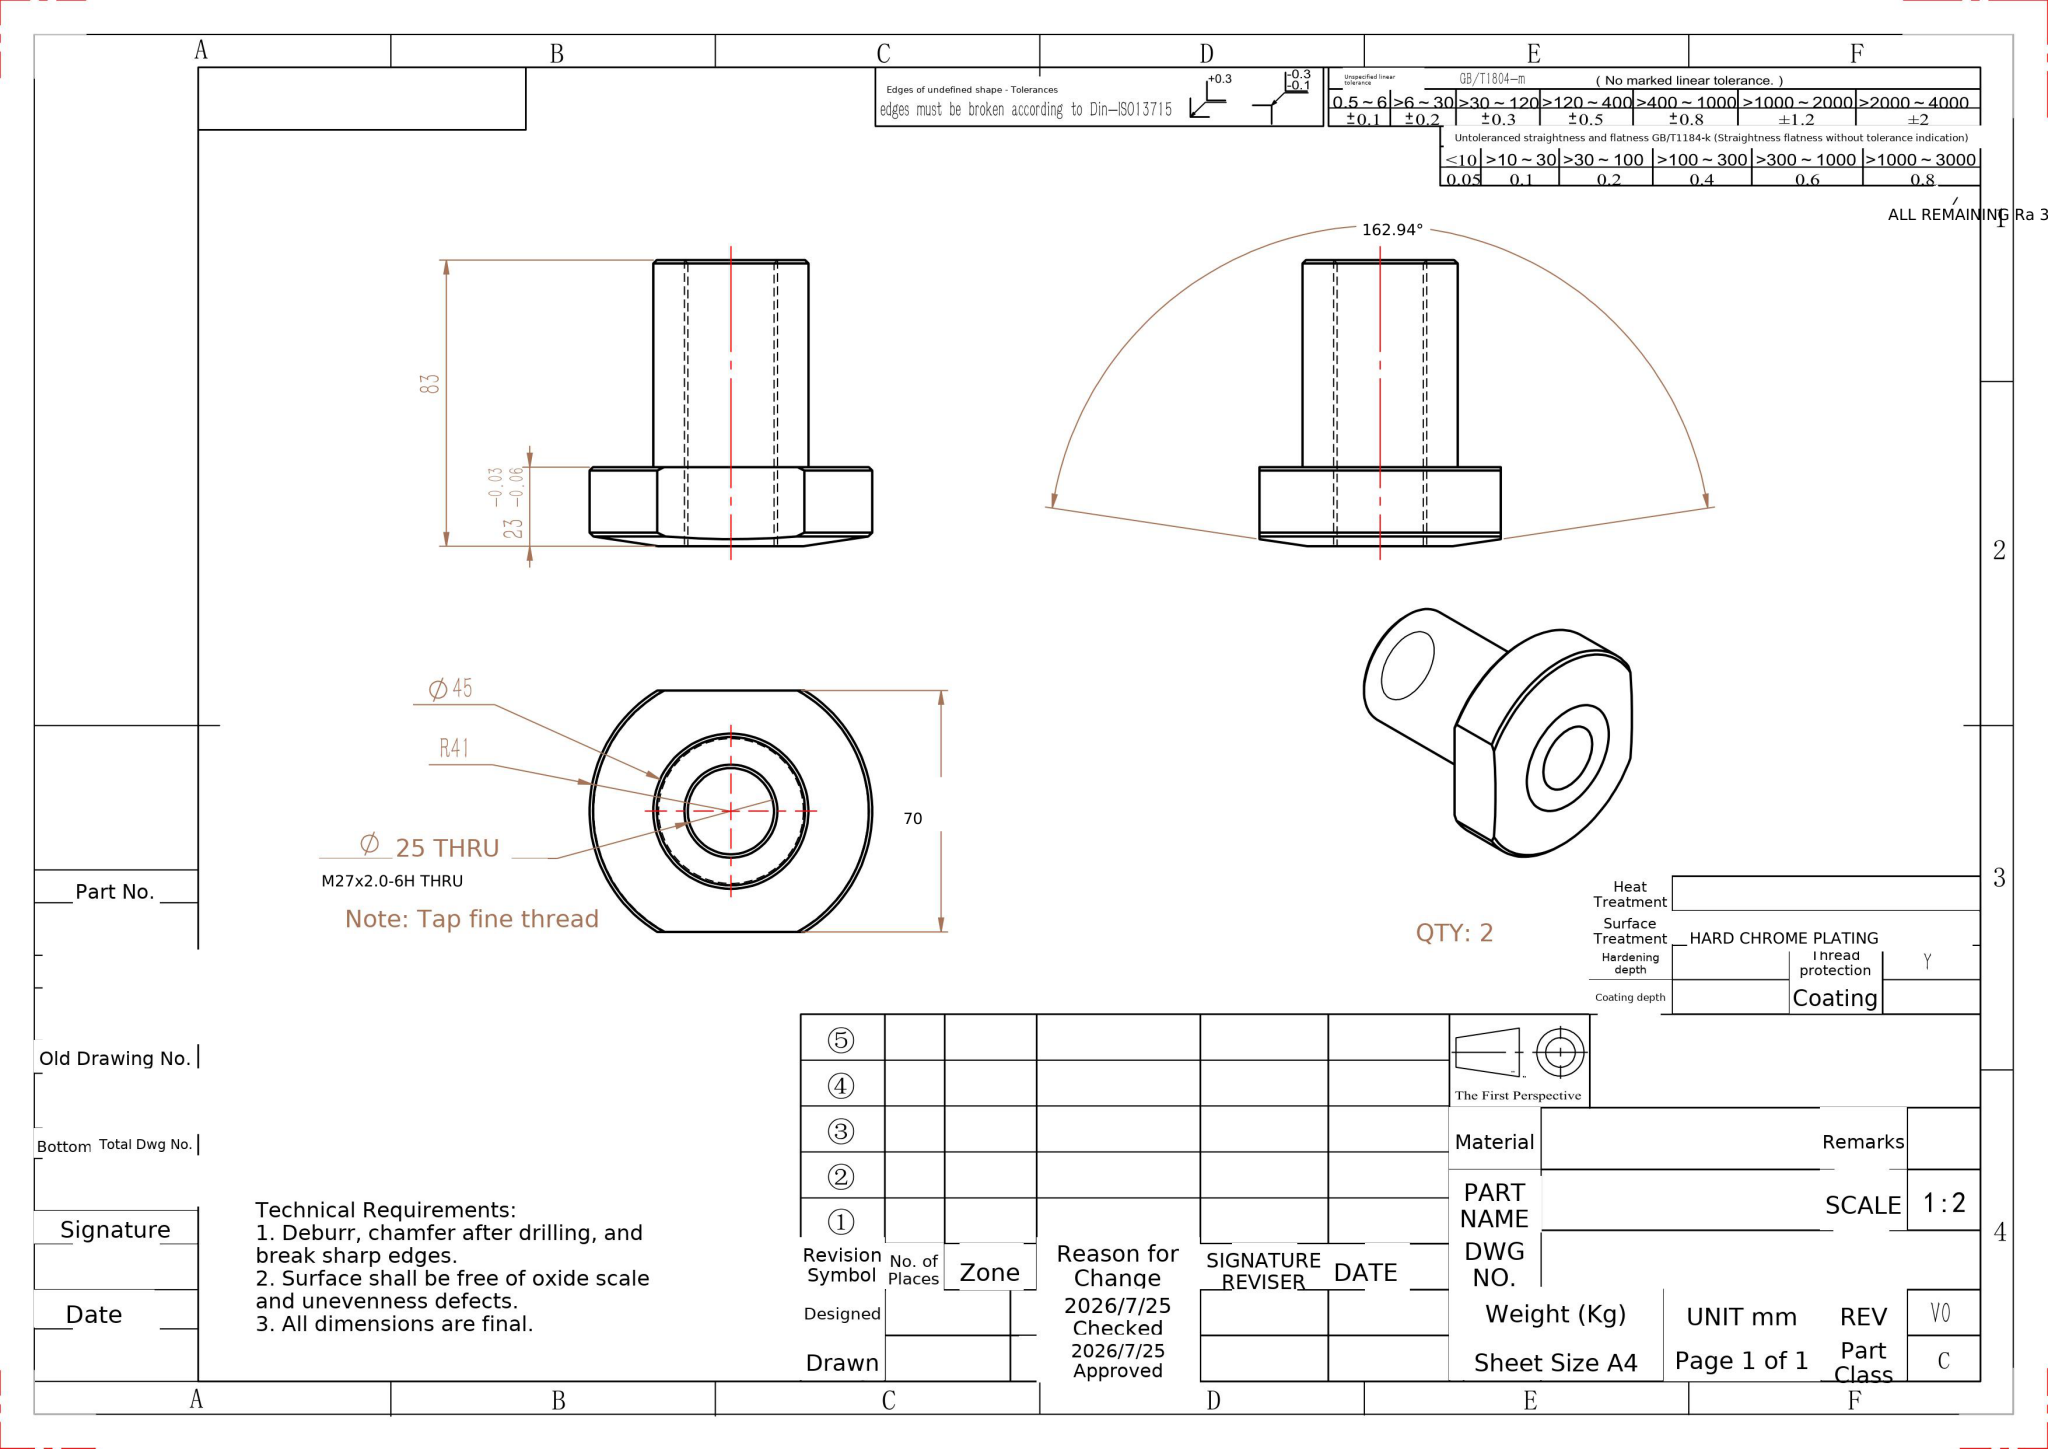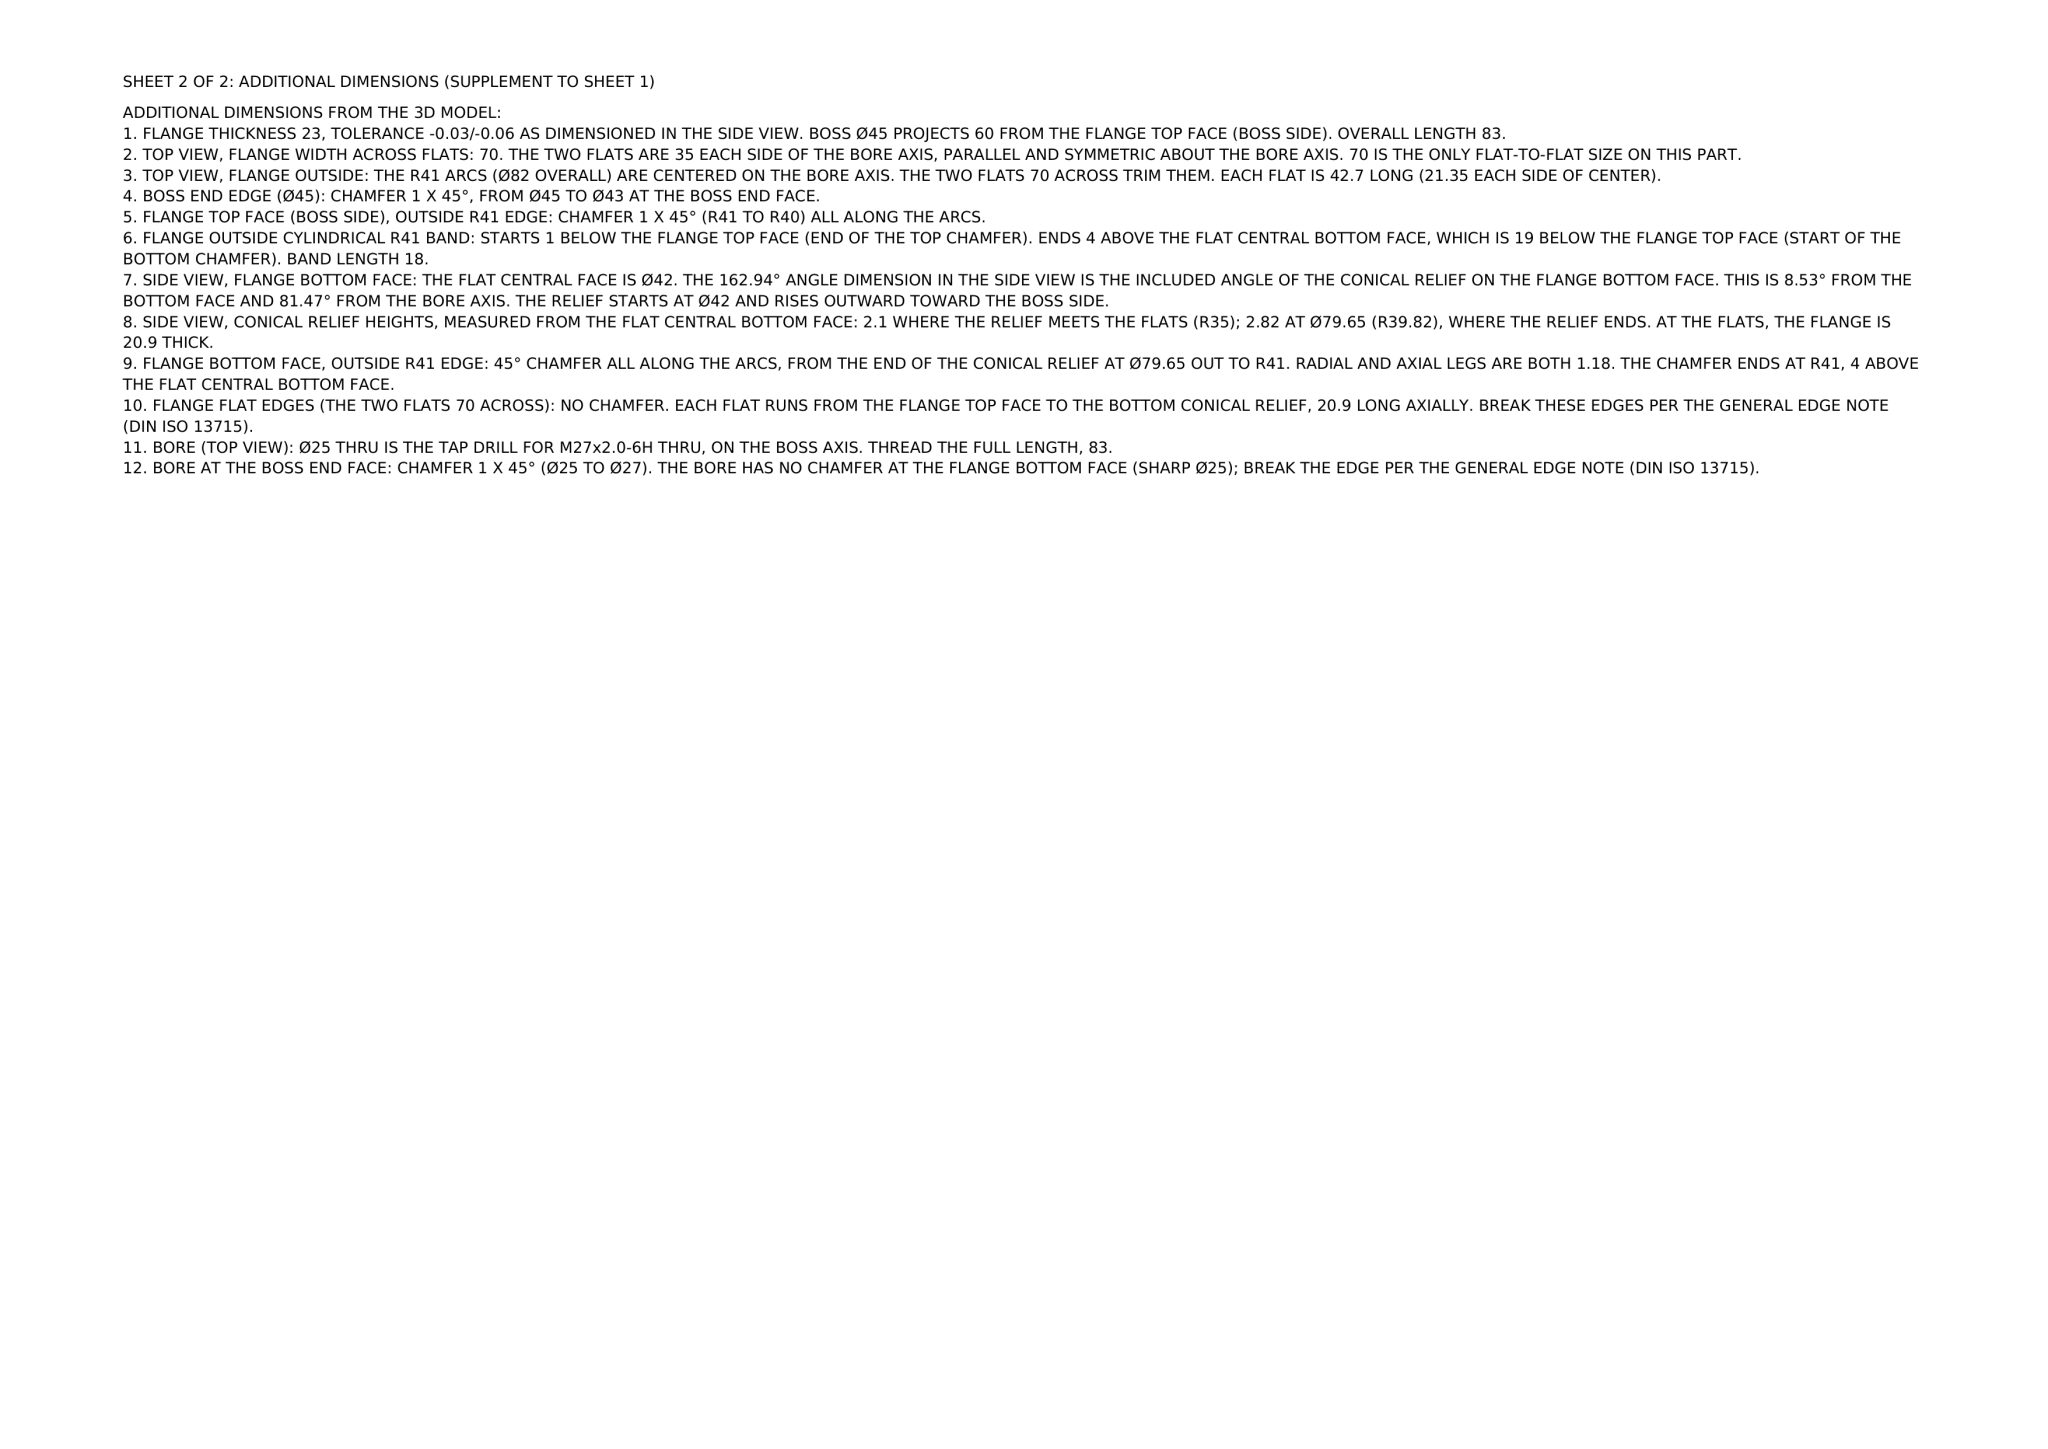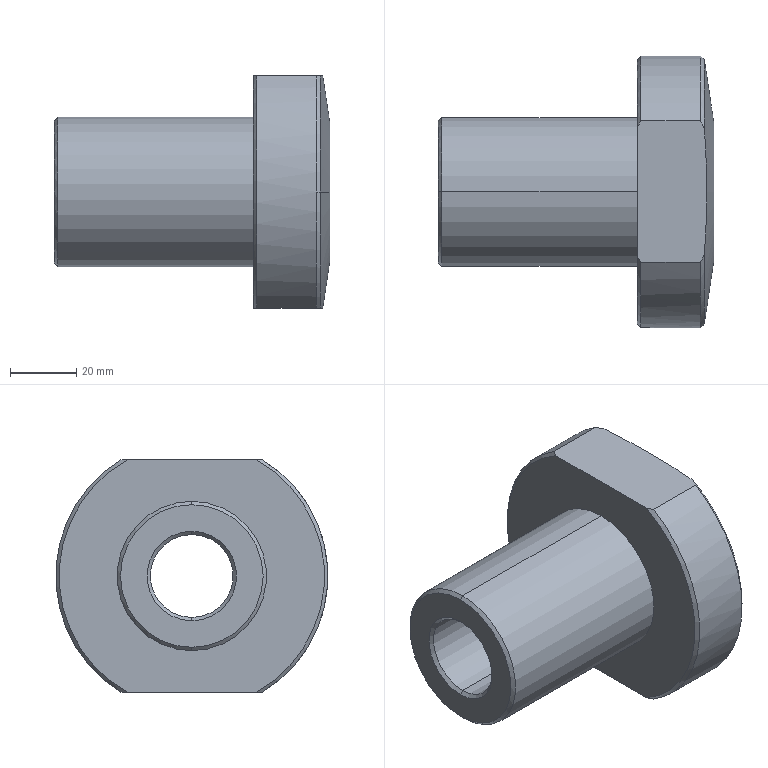Part | NX | mm | 1 solid | 22 faces | box 83 x 82 x 70 mm | volume 162318 mm3 | cone 11 | cylinder 6 | plane 5 | commonest cylinder face diameters 25 x2 45 x2 82 x2
STEP:
#1=CARTESIAN_POINT('',(23.176,-39.824,0.));
#2=VERTEX_POINT('',#1);
#3=CARTESIAN_POINT('',(23.176,-18.998,-35.));
#4=VERTEX_POINT('',#3);
#5=CARTESIAN_POINT('',(23.176,0.,0.));
#6=DIRECTION('',(1.,0.,0.));
#7=DIRECTION('',(-0.,1.,0.));
#8=AXIS2_PLACEMENT_3D('',#5,#6,#7);
#9=CIRCLE('',#8,39.824);
#10=EDGE_CURVE('',#2,#4,#9,.T.);
#11=ORIENTED_EDGE('',*,*,#10,.F.);
#12=CARTESIAN_POINT('',(22.,-41.,0.));
#13=VERTEX_POINT('',#12);
#14=CARTESIAN_POINT('',(23.176,-39.824,0.));
#15=DIRECTION('',(-0.7071,-0.7071,0.));
#16=VECTOR('',#15,1000.);
#17=LINE('',#14,#16);
#18=EDGE_CURVE('',#2,#13,#17,.T.);
#19=ORIENTED_EDGE('',*,*,#18,.T.);
#20=CARTESIAN_POINT('',(22.,-21.354,-35.));
#21=VERTEX_POINT('',#20);
#22=CARTESIAN_POINT('',(22.,0.,0.));
#23=DIRECTION('',(-1.,-0.,0.));
#24=DIRECTION('',(-0.,1.,0.));
#25=AXIS2_PLACEMENT_3D('',#22,#23,#24);
#26=CIRCLE('',#25,41.);
#27=EDGE_CURVE('',#21,#13,#26,.T.);
#28=ORIENTED_EDGE('',*,*,#27,.F.);
#29=CARTESIAN_POINT('',(23.176,-18.998,-35.));
#30=CARTESIAN_POINT('',(22.798,-19.79,-35.));
#31=CARTESIAN_POINT('',(22.406,-20.575,-35.));
#32=CARTESIAN_POINT('',(22.,-21.354,-35.));
#33=B_SPLINE_CURVE_WITH_KNOTS('',3,(#29,#30,#31,#32),.UNSPECIFIED.,.F.,.F.,(4,4),(0.,0.002634),.UNSPECIFIED.);
#34=EDGE_CURVE('',#4,#21,#33,.T.);
#35=ORIENTED_EDGE('',*,*,#34,.F.);
#36=EDGE_LOOP('',(#11,#19,#28,#35));
#37=FACE_OUTER_BOUND('',#36,.T.);
#38=CARTESIAN_POINT('',(23.176,0.,0.));
#39=DIRECTION('',(-1.,-0.,0.));
#40=DIRECTION('',(0.,-1.,0.));
#41=AXIS2_PLACEMENT_3D('',#38,#39,#40);
#42=CONICAL_SURFACE('',#41,39.824,0.7854);
#43=ADVANCED_FACE('',(#37),#42,.T.);
#44=CARTESIAN_POINT('',(-57.,0.,21.5));
#45=VERTEX_POINT('',#44);
#46=CARTESIAN_POINT('',(-57.,0.,-21.5));
#47=VERTEX_POINT('',#46);
#48=CARTESIAN_POINT('',(-57.,0.,0.));
#49=DIRECTION('',(-1.,0.,0.));
#50=DIRECTION('',(0.,0.,1.));
#51=AXIS2_PLACEMENT_3D('',#48,#49,#50);
#52=CIRCLE('',#51,21.5);
#53=EDGE_CURVE('',#45,#47,#52,.T.);
#54=ORIENTED_EDGE('',*,*,#53,.F.);
#55=CARTESIAN_POINT('',(-56.,0.,22.5));
#56=VERTEX_POINT('',#55);
#57=CARTESIAN_POINT('',(-57.,0.,21.5));
#58=DIRECTION('',(0.7071,0.,0.7071));
#59=VECTOR('',#58,1000.);
#60=LINE('',#57,#59);
#61=EDGE_CURVE('',#45,#56,#60,.T.);
#62=ORIENTED_EDGE('',*,*,#61,.T.);
#63=CARTESIAN_POINT('',(-56.,0.,-22.5));
#64=VERTEX_POINT('',#63);
#65=CARTESIAN_POINT('',(-56.,0.,0.));
#66=DIRECTION('',(1.,0.,0.));
#67=DIRECTION('',(0.,0.,1.));
#68=AXIS2_PLACEMENT_3D('',#65,#66,#67);
#69=CIRCLE('',#68,22.5);
#70=EDGE_CURVE('',#64,#56,#69,.T.);
#71=ORIENTED_EDGE('',*,*,#70,.F.);
#72=CARTESIAN_POINT('',(-57.,0.,-21.5));
#73=DIRECTION('',(0.7071,0.,-0.7071));
#74=VECTOR('',#73,1000.);
#75=LINE('',#72,#74);
#76=EDGE_CURVE('',#47,#64,#75,.T.);
#77=ORIENTED_EDGE('',*,*,#76,.F.);
#78=EDGE_LOOP('',(#54,#62,#71,#77));
#79=FACE_OUTER_BOUND('',#78,.T.);
#80=CARTESIAN_POINT('',(-57.,0.,0.));
#81=DIRECTION('',(1.,0.,0.));
#82=DIRECTION('',(0.,0.,-1.));
#83=AXIS2_PLACEMENT_3D('',#80,#81,#82);
#84=CONICAL_SURFACE('',#83,21.5,0.7854);
#85=ADVANCED_FACE('',(#79),#84,.T.);
#86=CARTESIAN_POINT('',(-56.,0.,-12.5));
#87=VERTEX_POINT('',#86);
#88=CARTESIAN_POINT('',(-56.,0.,12.5));
#89=VERTEX_POINT('',#88);
#90=CARTESIAN_POINT('',(-56.,0.,0.));
#91=DIRECTION('',(-1.,0.,0.));
#92=DIRECTION('',(0.,0.,1.));
#93=AXIS2_PLACEMENT_3D('',#90,#91,#92);
#94=CIRCLE('',#93,12.5);
#95=EDGE_CURVE('',#87,#89,#94,.T.);
#96=ORIENTED_EDGE('',*,*,#95,.F.);
#97=CARTESIAN_POINT('',(-57.,0.,-13.5));
#98=VERTEX_POINT('',#97);
#99=CARTESIAN_POINT('',(-56.,0.,-12.5));
#100=DIRECTION('',(-0.7071,0.,-0.7071));
#101=VECTOR('',#100,1000.);
#102=LINE('',#99,#101);
#103=EDGE_CURVE('',#87,#98,#102,.T.);
#104=ORIENTED_EDGE('',*,*,#103,.T.);
#105=CARTESIAN_POINT('',(-57.,0.,13.5));
#106=VERTEX_POINT('',#105);
#107=CARTESIAN_POINT('',(-57.,0.,0.));
#108=DIRECTION('',(1.,0.,0.));
#109=DIRECTION('',(0.,0.,1.));
#110=AXIS2_PLACEMENT_3D('',#107,#108,#109);
#111=CIRCLE('',#110,13.5);
#112=EDGE_CURVE('',#106,#98,#111,.T.);
#113=ORIENTED_EDGE('',*,*,#112,.F.);
#114=CARTESIAN_POINT('',(-56.,0.,12.5));
#115=DIRECTION('',(-0.7071,0.,0.7071));
#116=VECTOR('',#115,1000.);
#117=LINE('',#114,#116);
#118=EDGE_CURVE('',#89,#106,#117,.T.);
#119=ORIENTED_EDGE('',*,*,#118,.F.);
#120=EDGE_LOOP('',(#96,#104,#113,#119));
#121=FACE_OUTER_BOUND('',#120,.T.);
#122=CARTESIAN_POINT('',(-56.,0.,0.));
#123=DIRECTION('',(-1.,0.,0.));
#124=DIRECTION('',(0.,0.,1.));
#125=AXIS2_PLACEMENT_3D('',#122,#123,#124);
#126=CONICAL_SURFACE('',#125,12.5,0.7854);
#127=ADVANCED_FACE('',(#121),#126,.F.);
#128=CARTESIAN_POINT('',(26.,0.,-12.5));
#129=VERTEX_POINT('',#128);
#130=CARTESIAN_POINT('',(26.,0.,12.5));
#131=VERTEX_POINT('',#130);
#132=CARTESIAN_POINT('',(26.,0.,0.));
#133=DIRECTION('',(-1.,0.,0.));
#134=DIRECTION('',(0.,0.,1.));
#135=AXIS2_PLACEMENT_3D('',#132,#133,#134);
#136=CIRCLE('',#135,12.5);
#137=EDGE_CURVE('',#129,#131,#136,.T.);
#138=ORIENTED_EDGE('',*,*,#137,.F.);
#139=CARTESIAN_POINT('',(-57.,0.,-12.5));
#140=DIRECTION('',(-1.,0.,0.));
#141=VECTOR('',#140,1000.);
#142=LINE('',#139,#141);
#143=EDGE_CURVE('',#129,#87,#142,.T.);
#144=ORIENTED_EDGE('',*,*,#143,.T.);
#145=ORIENTED_EDGE('',*,*,#95,.T.);
#146=CARTESIAN_POINT('',(-57.,0.,12.5));
#147=DIRECTION('',(-1.,0.,0.));
#148=VECTOR('',#147,1000.);
#149=LINE('',#146,#148);
#150=EDGE_CURVE('',#131,#89,#149,.T.);
#151=ORIENTED_EDGE('',*,*,#150,.F.);
#152=EDGE_LOOP('',(#138,#144,#145,#151));
#153=FACE_OUTER_BOUND('',#152,.T.);
#154=CARTESIAN_POINT('',(-57.,0.,0.));
#155=DIRECTION('',(-1.,0.,0.));
#156=DIRECTION('',(0.,0.,1.));
#157=AXIS2_PLACEMENT_3D('',#154,#155,#156);
#158=CYLINDRICAL_SURFACE('',#157,12.5);
#159=ADVANCED_FACE('',(#153),#158,.F.);
#160=ORIENTED_EDGE('',*,*,#70,.T.);
#161=CARTESIAN_POINT('',(3.,0.,22.5));
#162=VERTEX_POINT('',#161);
#163=CARTESIAN_POINT('',(-57.,0.,22.5));
#164=DIRECTION('',(1.,0.,0.));
#165=VECTOR('',#164,1000.);
#166=LINE('',#163,#165);
#167=EDGE_CURVE('',#56,#162,#166,.T.);
#168=ORIENTED_EDGE('',*,*,#167,.T.);
#169=CARTESIAN_POINT('',(3.,0.,-22.5));
#170=VERTEX_POINT('',#169);
#171=CARTESIAN_POINT('',(3.,0.,0.));
#172=DIRECTION('',(-1.,0.,0.));
#173=DIRECTION('',(0.,0.,1.));
#174=AXIS2_PLACEMENT_3D('',#171,#172,#173);
#175=CIRCLE('',#174,22.5);
#176=EDGE_CURVE('',#162,#170,#175,.T.);
#177=ORIENTED_EDGE('',*,*,#176,.T.);
#178=CARTESIAN_POINT('',(-57.,0.,-22.5));
#179=DIRECTION('',(1.,0.,0.));
#180=VECTOR('',#179,1000.);
#181=LINE('',#178,#180);
#182=EDGE_CURVE('',#64,#170,#181,.T.);
#183=ORIENTED_EDGE('',*,*,#182,.F.);
#184=EDGE_LOOP('',(#160,#168,#177,#183));
#185=FACE_OUTER_BOUND('',#184,.T.);
#186=CARTESIAN_POINT('',(-57.,0.,0.));
#187=DIRECTION('',(1.,0.,0.));
#188=DIRECTION('',(0.,0.,-1.));
#189=AXIS2_PLACEMENT_3D('',#186,#187,#188);
#190=CYLINDRICAL_SURFACE('',#189,22.5);
#191=ADVANCED_FACE('',(#185),#190,.T.);
#192=CARTESIAN_POINT('',(26.,21.,0.));
#193=VERTEX_POINT('',#192);
#194=CARTESIAN_POINT('',(26.,-21.,0.));
#195=VERTEX_POINT('',#194);
#196=CARTESIAN_POINT('',(26.,0.,0.));
#197=DIRECTION('',(1.,0.,0.));
#198=DIRECTION('',(-0.,1.,0.));
#199=AXIS2_PLACEMENT_3D('',#196,#197,#198);
#200=CIRCLE('',#199,21.);
#201=EDGE_CURVE('',#193,#195,#200,.T.);
#202=ORIENTED_EDGE('',*,*,#201,.F.);
#203=CARTESIAN_POINT('',(23.176,39.824,0.));
#204=VERTEX_POINT('',#203);
#205=CARTESIAN_POINT('',(26.,21.,0.));
#206=DIRECTION('',(-0.1483,0.9889,0.));
#207=VECTOR('',#206,1000.);
#208=LINE('',#205,#207);
#209=EDGE_CURVE('',#193,#204,#208,.T.);
#210=ORIENTED_EDGE('',*,*,#209,.T.);
#211=CARTESIAN_POINT('',(23.176,18.998,35.));
#212=VERTEX_POINT('',#211);
#213=CARTESIAN_POINT('',(23.176,0.,0.));
#214=DIRECTION('',(1.,0.,0.));
#215=DIRECTION('',(-0.,1.,0.));
#216=AXIS2_PLACEMENT_3D('',#213,#214,#215);
#217=CIRCLE('',#216,39.824);
#218=EDGE_CURVE('',#204,#212,#217,.T.);
#219=ORIENTED_EDGE('',*,*,#218,.T.);
#220=CARTESIAN_POINT('',(23.176,-18.998,35.));
#221=VERTEX_POINT('',#220);
#222=CARTESIAN_POINT('',(23.176,18.998,35.));
#223=CARTESIAN_POINT('',(23.402,15.846,35.));
#224=CARTESIAN_POINT('',(23.584,12.691,35.));
#225=CARTESIAN_POINT('',(23.833,6.372,35.));
#226=CARTESIAN_POINT('',(23.899,3.208,35.));
#227=CARTESIAN_POINT('',(23.901,-3.129,35.));
#228=CARTESIAN_POINT('',(23.835,-6.303,35.));
#229=CARTESIAN_POINT('',(23.586,-12.659,35.));
#230=CARTESIAN_POINT('',(23.403,-15.83,35.));
#231=CARTESIAN_POINT('',(23.176,-18.998,35.));
#232=B_SPLINE_CURVE_WITH_KNOTS('',3,(#222,#223,#224,#225,#226,#227,#228,#229,#230,#231),.UNSPECIFIED.,.F.,.F.,(4,2,2,2,4),(0.04542,0.0549,0.06438,0.07386,0.08334),.UNSPECIFIED.);
#233=EDGE_CURVE('',#212,#221,#232,.T.);
#234=ORIENTED_EDGE('',*,*,#233,.T.);
#235=CARTESIAN_POINT('',(23.176,0.,0.));
#236=DIRECTION('',(1.,0.,0.));
#237=DIRECTION('',(-0.,1.,0.));
#238=AXIS2_PLACEMENT_3D('',#235,#236,#237);
#239=CIRCLE('',#238,39.824);
#240=EDGE_CURVE('',#221,#2,#239,.T.);
#241=ORIENTED_EDGE('',*,*,#240,.T.);
#242=CARTESIAN_POINT('',(26.,-21.,0.));
#243=DIRECTION('',(-0.1483,-0.9889,0.));
#244=VECTOR('',#243,1000.);
#245=LINE('',#242,#244);
#246=EDGE_CURVE('',#195,#2,#245,.T.);
#247=ORIENTED_EDGE('',*,*,#246,.F.);
#248=EDGE_LOOP('',(#202,#210,#219,#234,#241,#247));
#249=FACE_OUTER_BOUND('',#248,.T.);
#250=CARTESIAN_POINT('',(26.,0.,0.));
#251=DIRECTION('',(-1.,-0.,0.));
#252=DIRECTION('',(0.,-1.,0.));
#253=AXIS2_PLACEMENT_3D('',#250,#251,#252);
#254=CONICAL_SURFACE('',#253,21.,1.422);
#255=ADVANCED_FACE('',(#249),#254,.T.);
#256=CARTESIAN_POINT('',(22.,21.354,35.));
#257=VERTEX_POINT('',#256);
#258=CARTESIAN_POINT('',(4.,21.354,35.));
#259=VERTEX_POINT('',#258);
#260=CARTESIAN_POINT('',(141.966,21.354,35.));
#261=DIRECTION('',(-1.,0.,0.));
#262=VECTOR('',#261,1000.);
#263=LINE('',#260,#262);
#264=EDGE_CURVE('',#257,#259,#263,.T.);
#265=ORIENTED_EDGE('',*,*,#264,.F.);
#266=CARTESIAN_POINT('',(22.,21.354,-35.));
#267=VERTEX_POINT('',#266);
#268=CARTESIAN_POINT('',(22.,0.,0.));
#269=DIRECTION('',(-1.,-0.,0.));
#270=DIRECTION('',(-0.,1.,0.));
#271=AXIS2_PLACEMENT_3D('',#268,#269,#270);
#272=CIRCLE('',#271,41.);
#273=EDGE_CURVE('',#257,#267,#272,.T.);
#274=ORIENTED_EDGE('',*,*,#273,.T.);
#275=CARTESIAN_POINT('',(4.,21.354,-35.));
#276=VERTEX_POINT('',#275);
#277=CARTESIAN_POINT('',(141.966,21.354,-35.));
#278=DIRECTION('',(1.,0.,0.));
#279=VECTOR('',#278,1000.);
#280=LINE('',#277,#279);
#281=EDGE_CURVE('',#276,#267,#280,.T.);
#282=ORIENTED_EDGE('',*,*,#281,.F.);
#283=CARTESIAN_POINT('',(4.,0.,0.));
#284=DIRECTION('',(1.,0.,0.));
#285=DIRECTION('',(0.,-0.,1.));
#286=AXIS2_PLACEMENT_3D('',#283,#284,#285);
#287=CIRCLE('',#286,41.);
#288=EDGE_CURVE('',#276,#259,#287,.T.);
#289=ORIENTED_EDGE('',*,*,#288,.T.);
#290=EDGE_LOOP('',(#265,#274,#282,#289));
#291=FACE_OUTER_BOUND('',#290,.T.);
#292=CARTESIAN_POINT('',(141.966,0.,0.));
#293=DIRECTION('',(-1.,0.,0.));
#294=DIRECTION('',(0.,0.,1.));
#295=AXIS2_PLACEMENT_3D('',#292,#293,#294);
#296=CYLINDRICAL_SURFACE('',#295,41.);
#297=ADVANCED_FACE('',(#291),#296,.T.);
#298=CARTESIAN_POINT('',(4.,-21.354,-35.));
#299=VERTEX_POINT('',#298);
#300=CARTESIAN_POINT('',(141.966,-21.354,-35.));
#301=DIRECTION('',(-1.,0.,0.));
#302=VECTOR('',#301,1000.);
#303=LINE('',#300,#302);
#304=EDGE_CURVE('',#21,#299,#303,.T.);
#305=ORIENTED_EDGE('',*,*,#304,.F.);
#306=ORIENTED_EDGE('',*,*,#27,.T.);
#307=CARTESIAN_POINT('',(22.,-21.354,35.));
#308=VERTEX_POINT('',#307);
#309=CARTESIAN_POINT('',(22.,0.,0.));
#310=DIRECTION('',(-1.,-0.,0.));
#311=DIRECTION('',(-0.,1.,0.));
#312=AXIS2_PLACEMENT_3D('',#309,#310,#311);
#313=CIRCLE('',#312,41.);
#314=EDGE_CURVE('',#13,#308,#313,.T.);
#315=ORIENTED_EDGE('',*,*,#314,.T.);
#316=CARTESIAN_POINT('',(4.,-21.354,35.));
#317=VERTEX_POINT('',#316);
#318=CARTESIAN_POINT('',(141.966,-21.354,35.));
#319=DIRECTION('',(1.,0.,0.));
#320=VECTOR('',#319,1000.);
#321=LINE('',#318,#320);
#322=EDGE_CURVE('',#317,#308,#321,.T.);
#323=ORIENTED_EDGE('',*,*,#322,.F.);
#324=CARTESIAN_POINT('',(4.,0.,0.));
#325=DIRECTION('',(1.,0.,0.));
#326=DIRECTION('',(0.,0.,1.));
#327=AXIS2_PLACEMENT_3D('',#324,#325,#326);
#328=CIRCLE('',#327,41.);
#329=EDGE_CURVE('',#317,#299,#328,.T.);
#330=ORIENTED_EDGE('',*,*,#329,.T.);
#331=EDGE_LOOP('',(#305,#306,#315,#323,#330));
#332=FACE_OUTER_BOUND('',#331,.T.);
#333=CARTESIAN_POINT('',(141.966,0.,0.));
#334=DIRECTION('',(-1.,0.,0.));
#335=DIRECTION('',(0.,0.,1.));
#336=AXIS2_PLACEMENT_3D('',#333,#334,#335);
#337=CYLINDRICAL_SURFACE('',#336,41.);
#338=ADVANCED_FACE('',(#332),#337,.T.);
#339=ORIENTED_EDGE('',*,*,#233,.F.);
#340=CARTESIAN_POINT('',(23.176,18.998,35.));
#341=CARTESIAN_POINT('',(22.798,19.79,35.));
#342=CARTESIAN_POINT('',(22.406,20.575,35.));
#343=CARTESIAN_POINT('',(22.,21.354,35.));
#344=B_SPLINE_CURVE_WITH_KNOTS('',3,(#340,#341,#342,#343),.UNSPECIFIED.,.F.,.F.,(4,4),(0.,0.002634),.UNSPECIFIED.);
#345=EDGE_CURVE('',#212,#257,#344,.T.);
#346=ORIENTED_EDGE('',*,*,#345,.T.);
#347=ORIENTED_EDGE('',*,*,#264,.T.);
#348=CARTESIAN_POINT('',(3.,19.365,35.));
#349=VERTEX_POINT('',#348);
#350=CARTESIAN_POINT('',(4.,21.354,35.));
#351=CARTESIAN_POINT('',(3.657,20.696,35.));
#352=CARTESIAN_POINT('',(3.323,20.033,35.));
#353=CARTESIAN_POINT('',(3.,19.365,35.));
#354=B_SPLINE_CURVE_WITH_KNOTS('',3,(#350,#351,#352,#353),.UNSPECIFIED.,.F.,.F.,(4,4),(0.,0.002226),.UNSPECIFIED.);
#355=EDGE_CURVE('',#259,#349,#354,.T.);
#356=ORIENTED_EDGE('',*,*,#355,.T.);
#357=CARTESIAN_POINT('',(3.,-19.365,35.));
#358=VERTEX_POINT('',#357);
#359=CARTESIAN_POINT('',(3.,45.286,35.));
#360=DIRECTION('',(0.,-1.,0.));
#361=VECTOR('',#360,1000.);
#362=LINE('',#359,#361);
#363=EDGE_CURVE('',#349,#358,#362,.T.);
#364=ORIENTED_EDGE('',*,*,#363,.T.);
#365=CARTESIAN_POINT('',(3.,-19.365,35.));
#366=CARTESIAN_POINT('',(3.323,-20.033,35.));
#367=CARTESIAN_POINT('',(3.657,-20.696,35.));
#368=CARTESIAN_POINT('',(4.,-21.354,35.));
#369=B_SPLINE_CURVE_WITH_KNOTS('',3,(#365,#366,#367,#368),.UNSPECIFIED.,.F.,.F.,(4,4),(0.,0.002226),.UNSPECIFIED.);
#370=EDGE_CURVE('',#358,#317,#369,.T.);
#371=ORIENTED_EDGE('',*,*,#370,.T.);
#372=ORIENTED_EDGE('',*,*,#322,.T.);
#373=CARTESIAN_POINT('',(22.,-21.354,35.));
#374=CARTESIAN_POINT('',(22.406,-20.575,35.));
#375=CARTESIAN_POINT('',(22.798,-19.79,35.));
#376=CARTESIAN_POINT('',(23.176,-18.998,35.));
#377=B_SPLINE_CURVE_WITH_KNOTS('',3,(#373,#374,#375,#376),.UNSPECIFIED.,.F.,.F.,(4,4),(0.,0.002634),.UNSPECIFIED.);
#378=EDGE_CURVE('',#308,#221,#377,.T.);
#379=ORIENTED_EDGE('',*,*,#378,.T.);
#380=EDGE_LOOP('',(#339,#346,#347,#356,#364,#371,#372,#379));
#381=FACE_OUTER_BOUND('',#380,.T.);
#382=CARTESIAN_POINT('',(26.,45.286,35.));
#383=DIRECTION('',(0.,-0.,-1.));
#384=DIRECTION('',(0.,1.,-0.));
#385=AXIS2_PLACEMENT_3D('',#382,#383,#384);
#386=PLANE('',#385);
#387=ADVANCED_FACE('',(#381),#386,.F.);
#388=ORIENTED_EDGE('',*,*,#281,.T.);
#389=CARTESIAN_POINT('',(23.176,18.998,-35.));
#390=VERTEX_POINT('',#389);
#391=CARTESIAN_POINT('',(22.,21.354,-35.));
#392=CARTESIAN_POINT('',(22.406,20.575,-35.));
#393=CARTESIAN_POINT('',(22.798,19.79,-35.));
#394=CARTESIAN_POINT('',(23.176,18.998,-35.));
#395=B_SPLINE_CURVE_WITH_KNOTS('',3,(#391,#392,#393,#394),.UNSPECIFIED.,.F.,.F.,(4,4),(0.,0.002634),.UNSPECIFIED.);
#396=EDGE_CURVE('',#267,#390,#395,.T.);
#397=ORIENTED_EDGE('',*,*,#396,.T.);
#398=CARTESIAN_POINT('',(23.176,-18.998,-35.));
#399=CARTESIAN_POINT('',(23.402,-15.846,-35.));
#400=CARTESIAN_POINT('',(23.584,-12.691,-35.));
#401=CARTESIAN_POINT('',(23.833,-6.372,-35.));
#402=CARTESIAN_POINT('',(23.899,-3.208,-35.));
#403=CARTESIAN_POINT('',(23.901,3.129,-35.));
#404=CARTESIAN_POINT('',(23.835,6.303,-35.));
#405=CARTESIAN_POINT('',(23.586,12.659,-35.));
#406=CARTESIAN_POINT('',(23.403,15.83,-35.));
#407=CARTESIAN_POINT('',(23.176,18.998,-35.));
#408=B_SPLINE_CURVE_WITH_KNOTS('',3,(#398,#399,#400,#401,#402,#403,#404,#405,#406,#407),.UNSPECIFIED.,.F.,.F.,(4,2,2,2,4),(0.04542,0.0549,0.06438,0.07386,0.08334),.UNSPECIFIED.);
#409=EDGE_CURVE('',#4,#390,#408,.T.);
#410=ORIENTED_EDGE('',*,*,#409,.F.);
#411=ORIENTED_EDGE('',*,*,#34,.T.);
#412=ORIENTED_EDGE('',*,*,#304,.T.);
#413=CARTESIAN_POINT('',(3.,-19.365,-35.));
#414=VERTEX_POINT('',#413);
#415=CARTESIAN_POINT('',(4.,-21.354,-35.));
#416=CARTESIAN_POINT('',(3.657,-20.696,-35.));
#417=CARTESIAN_POINT('',(3.323,-20.033,-35.));
#418=CARTESIAN_POINT('',(3.,-19.365,-35.));
#419=B_SPLINE_CURVE_WITH_KNOTS('',3,(#415,#416,#417,#418),.UNSPECIFIED.,.F.,.F.,(4,4),(0.,0.002226),.UNSPECIFIED.);
#420=EDGE_CURVE('',#299,#414,#419,.T.);
#421=ORIENTED_EDGE('',*,*,#420,.T.);
#422=CARTESIAN_POINT('',(3.,19.365,-35.));
#423=VERTEX_POINT('',#422);
#424=CARTESIAN_POINT('',(3.,43.028,-35.));
#425=DIRECTION('',(0.,1.,-0.));
#426=VECTOR('',#425,1000.);
#427=LINE('',#424,#426);
#428=EDGE_CURVE('',#414,#423,#427,.T.);
#429=ORIENTED_EDGE('',*,*,#428,.T.);
#430=CARTESIAN_POINT('',(3.,19.365,-35.));
#431=CARTESIAN_POINT('',(3.323,20.033,-35.));
#432=CARTESIAN_POINT('',(3.657,20.696,-35.));
#433=CARTESIAN_POINT('',(4.,21.354,-35.));
#434=B_SPLINE_CURVE_WITH_KNOTS('',3,(#430,#431,#432,#433),.UNSPECIFIED.,.F.,.F.,(4,4),(0.,0.002226),.UNSPECIFIED.);
#435=EDGE_CURVE('',#423,#276,#434,.T.);
#436=ORIENTED_EDGE('',*,*,#435,.T.);
#437=EDGE_LOOP('',(#388,#397,#410,#411,#412,#421,#429,#436));
#438=FACE_OUTER_BOUND('',#437,.T.);
#439=CARTESIAN_POINT('',(26.,43.028,-35.));
#440=DIRECTION('',(0.,0.,1.));
#441=DIRECTION('',(0.,-1.,0.));
#442=AXIS2_PLACEMENT_3D('',#439,#440,#441);
#443=PLANE('',#442);
#444=ADVANCED_FACE('',(#438),#443,.F.);
#445=CARTESIAN_POINT('',(3.,0.,0.));
#446=DIRECTION('',(-1.,0.,0.));
#447=DIRECTION('',(0.,0.,1.));
#448=AXIS2_PLACEMENT_3D('',#445,#446,#447);
#449=CIRCLE('',#448,22.5);
#450=EDGE_CURVE('',#170,#162,#449,.T.);
#451=ORIENTED_EDGE('',*,*,#450,.F.);
#452=ORIENTED_EDGE('',*,*,#176,.F.);
#453=EDGE_LOOP('',(#451,#452));
#454=FACE_BOUND('',#453,.T.);
#455=ORIENTED_EDGE('',*,*,#428,.F.);
#456=CARTESIAN_POINT('',(3.,0.,0.));
#457=DIRECTION('',(-1.,0.,0.));
#458=DIRECTION('',(0.,0.,1.));
#459=AXIS2_PLACEMENT_3D('',#456,#457,#458);
#460=CIRCLE('',#459,40.);
#461=EDGE_CURVE('',#414,#358,#460,.T.);
#462=ORIENTED_EDGE('',*,*,#461,.T.);
#463=ORIENTED_EDGE('',*,*,#363,.F.);
#464=CARTESIAN_POINT('',(3.,0.,0.));
#465=DIRECTION('',(-1.,0.,0.));
#466=DIRECTION('',(0.,0.,1.));
#467=AXIS2_PLACEMENT_3D('',#464,#465,#466);
#468=CIRCLE('',#467,40.);
#469=EDGE_CURVE('',#349,#423,#468,.T.);
#470=ORIENTED_EDGE('',*,*,#469,.T.);
#471=EDGE_LOOP('',(#455,#462,#463,#470));
#472=FACE_OUTER_BOUND('',#471,.T.);
#473=CARTESIAN_POINT('',(3.,26.5,0.));
#474=DIRECTION('',(-1.,0.,0.));
#475=DIRECTION('',(0.,0.,1.));
#476=AXIS2_PLACEMENT_3D('',#473,#474,#475);
#477=PLANE('',#476);
#478=ADVANCED_FACE('',(#454,#472),#477,.T.);
#479=ORIENTED_EDGE('',*,*,#209,.F.);
#480=CARTESIAN_POINT('',(26.,0.,0.));
#481=DIRECTION('',(1.,0.,0.));
#482=DIRECTION('',(-0.,1.,0.));
#483=AXIS2_PLACEMENT_3D('',#480,#481,#482);
#484=CIRCLE('',#483,21.);
#485=EDGE_CURVE('',#195,#193,#484,.T.);
#486=ORIENTED_EDGE('',*,*,#485,.F.);
#487=ORIENTED_EDGE('',*,*,#246,.T.);
#488=ORIENTED_EDGE('',*,*,#10,.T.);
#489=ORIENTED_EDGE('',*,*,#409,.T.);
#490=CARTESIAN_POINT('',(23.176,0.,0.));
#491=DIRECTION('',(1.,0.,0.));
#492=DIRECTION('',(-0.,1.,0.));
#493=AXIS2_PLACEMENT_3D('',#490,#491,#492);
#494=CIRCLE('',#493,39.824);
#495=EDGE_CURVE('',#390,#204,#494,.T.);
#496=ORIENTED_EDGE('',*,*,#495,.T.);
#497=EDGE_LOOP('',(#479,#486,#487,#488,#489,#496));
#498=FACE_OUTER_BOUND('',#497,.T.);
#499=CARTESIAN_POINT('',(26.,0.,0.));
#500=DIRECTION('',(-1.,-0.,0.));
#501=DIRECTION('',(0.,-1.,0.));
#502=AXIS2_PLACEMENT_3D('',#499,#500,#501);
#503=CONICAL_SURFACE('',#502,21.,1.422);
#504=ADVANCED_FACE('',(#498),#503,.T.);
#505=CARTESIAN_POINT('',(26.,0.,0.));
#506=DIRECTION('',(-1.,0.,0.));
#507=DIRECTION('',(0.,0.,1.));
#508=AXIS2_PLACEMENT_3D('',#505,#506,#507);
#509=CIRCLE('',#508,12.5);
#510=EDGE_CURVE('',#131,#129,#509,.T.);
#511=ORIENTED_EDGE('',*,*,#510,.T.);
#512=ORIENTED_EDGE('',*,*,#137,.T.);
#513=EDGE_LOOP('',(#511,#512));
#514=FACE_BOUND('',#513,.T.);
#515=ORIENTED_EDGE('',*,*,#485,.T.);
#516=ORIENTED_EDGE('',*,*,#201,.T.);
#517=EDGE_LOOP('',(#515,#516));
#518=FACE_OUTER_BOUND('',#517,.T.);
#519=CARTESIAN_POINT('',(26.,13.,0.));
#520=DIRECTION('',(1.,0.,0.));
#521=DIRECTION('',(0.,0.,-1.));
#522=AXIS2_PLACEMENT_3D('',#519,#520,#521);
#523=PLANE('',#522);
#524=ADVANCED_FACE('',(#514,#518),#523,.T.);
#525=ORIENTED_EDGE('',*,*,#167,.F.);
#526=CARTESIAN_POINT('',(-56.,0.,0.));
#527=DIRECTION('',(1.,0.,0.));
#528=DIRECTION('',(0.,0.,1.));
#529=AXIS2_PLACEMENT_3D('',#526,#527,#528);
#530=CIRCLE('',#529,22.5);
#531=EDGE_CURVE('',#56,#64,#530,.T.);
#532=ORIENTED_EDGE('',*,*,#531,.T.);
#533=ORIENTED_EDGE('',*,*,#182,.T.);
#534=ORIENTED_EDGE('',*,*,#450,.T.);
#535=EDGE_LOOP('',(#525,#532,#533,#534));
#536=FACE_OUTER_BOUND('',#535,.T.);
#537=CARTESIAN_POINT('',(-57.,0.,0.));
#538=DIRECTION('',(1.,0.,0.));
#539=DIRECTION('',(0.,0.,-1.));
#540=AXIS2_PLACEMENT_3D('',#537,#538,#539);
#541=CYLINDRICAL_SURFACE('',#540,22.5);
#542=ADVANCED_FACE('',(#536),#541,.T.);
#543=ORIENTED_EDGE('',*,*,#112,.T.);
#544=CARTESIAN_POINT('',(-57.,0.,0.));
#545=DIRECTION('',(1.,0.,0.));
#546=DIRECTION('',(0.,0.,1.));
#547=AXIS2_PLACEMENT_3D('',#544,#545,#546);
#548=CIRCLE('',#547,13.5);
#549=EDGE_CURVE('',#98,#106,#548,.T.);
#550=ORIENTED_EDGE('',*,*,#549,.T.);
#551=EDGE_LOOP('',(#543,#550));
#552=FACE_BOUND('',#551,.T.);
#553=CARTESIAN_POINT('',(-57.,0.,0.));
#554=DIRECTION('',(-1.,0.,0.));
#555=DIRECTION('',(0.,0.,1.));
#556=AXIS2_PLACEMENT_3D('',#553,#554,#555);
#557=CIRCLE('',#556,21.5);
#558=EDGE_CURVE('',#47,#45,#557,.T.);
#559=ORIENTED_EDGE('',*,*,#558,.T.);
#560=ORIENTED_EDGE('',*,*,#53,.T.);
#561=EDGE_LOOP('',(#559,#560));
#562=FACE_OUTER_BOUND('',#561,.T.);
#563=CARTESIAN_POINT('',(-57.,0.,0.));
#564=DIRECTION('',(-1.,0.,0.));
#565=DIRECTION('',(0.,0.,1.));
#566=AXIS2_PLACEMENT_3D('',#563,#564,#565);
#567=PLANE('',#566);
#568=ADVANCED_FACE('',(#552,#562),#567,.T.);
#569=ORIENTED_EDGE('',*,*,#143,.F.);
#570=ORIENTED_EDGE('',*,*,#510,.F.);
#571=ORIENTED_EDGE('',*,*,#150,.T.);
#572=CARTESIAN_POINT('',(-56.,0.,0.));
#573=DIRECTION('',(-1.,0.,0.));
#574=DIRECTION('',(0.,0.,1.));
#575=AXIS2_PLACEMENT_3D('',#572,#573,#574);
#576=CIRCLE('',#575,12.5);
#577=EDGE_CURVE('',#89,#87,#576,.T.);
#578=ORIENTED_EDGE('',*,*,#577,.T.);
#579=EDGE_LOOP('',(#569,#570,#571,#578));
#580=FACE_OUTER_BOUND('',#579,.T.);
#581=CARTESIAN_POINT('',(-57.,0.,0.));
#582=DIRECTION('',(-1.,0.,0.));
#583=DIRECTION('',(0.,0.,1.));
#584=AXIS2_PLACEMENT_3D('',#581,#582,#583);
#585=CYLINDRICAL_SURFACE('',#584,12.5);
#586=ADVANCED_FACE('',(#580),#585,.F.);
#587=ORIENTED_EDGE('',*,*,#103,.F.);
#588=ORIENTED_EDGE('',*,*,#577,.F.);
#589=ORIENTED_EDGE('',*,*,#118,.T.);
#590=ORIENTED_EDGE('',*,*,#549,.F.);
#591=EDGE_LOOP('',(#587,#588,#589,#590));
#592=FACE_OUTER_BOUND('',#591,.T.);
#593=CARTESIAN_POINT('',(-56.,0.,0.));
#594=DIRECTION('',(-1.,0.,0.));
#595=DIRECTION('',(0.,0.,1.));
#596=AXIS2_PLACEMENT_3D('',#593,#594,#595);
#597=CONICAL_SURFACE('',#596,12.5,0.7854);
#598=ADVANCED_FACE('',(#592),#597,.F.);
#599=ORIENTED_EDGE('',*,*,#61,.F.);
#600=ORIENTED_EDGE('',*,*,#558,.F.);
#601=ORIENTED_EDGE('',*,*,#76,.T.);
#602=ORIENTED_EDGE('',*,*,#531,.F.);
#603=EDGE_LOOP('',(#599,#600,#601,#602));
#604=FACE_OUTER_BOUND('',#603,.T.);
#605=CARTESIAN_POINT('',(-57.,0.,0.));
#606=DIRECTION('',(1.,0.,0.));
#607=DIRECTION('',(0.,0.,-1.));
#608=AXIS2_PLACEMENT_3D('',#605,#606,#607);
#609=CONICAL_SURFACE('',#608,21.5,0.7854);
#610=ADVANCED_FACE('',(#604),#609,.T.);
#611=ORIENTED_EDGE('',*,*,#396,.F.);
#612=ORIENTED_EDGE('',*,*,#273,.F.);
#613=ORIENTED_EDGE('',*,*,#345,.F.);
#614=ORIENTED_EDGE('',*,*,#218,.F.);
#615=ORIENTED_EDGE('',*,*,#495,.F.);
#616=EDGE_LOOP('',(#611,#612,#613,#614,#615));
#617=FACE_OUTER_BOUND('',#616,.T.);
#618=CARTESIAN_POINT('',(23.176,0.,0.));
#619=DIRECTION('',(-1.,-0.,0.));
#620=DIRECTION('',(0.,-1.,0.));
#621=AXIS2_PLACEMENT_3D('',#618,#619,#620);
#622=CONICAL_SURFACE('',#621,39.824,0.7854);
#623=ADVANCED_FACE('',(#617),#622,.T.);
#624=ORIENTED_EDGE('',*,*,#18,.F.);
#625=ORIENTED_EDGE('',*,*,#240,.F.);
#626=ORIENTED_EDGE('',*,*,#378,.F.);
#627=ORIENTED_EDGE('',*,*,#314,.F.);
#628=EDGE_LOOP('',(#624,#625,#626,#627));
#629=FACE_OUTER_BOUND('',#628,.T.);
#630=CARTESIAN_POINT('',(23.176,0.,0.));
#631=DIRECTION('',(-1.,-0.,0.));
#632=DIRECTION('',(0.,-1.,0.));
#633=AXIS2_PLACEMENT_3D('',#630,#631,#632);
#634=CONICAL_SURFACE('',#633,39.824,0.7854);
#635=ADVANCED_FACE('',(#629),#634,.T.);
#636=ORIENTED_EDGE('',*,*,#420,.F.);
#637=ORIENTED_EDGE('',*,*,#329,.F.);
#638=ORIENTED_EDGE('',*,*,#370,.F.);
#639=ORIENTED_EDGE('',*,*,#461,.F.);
#640=EDGE_LOOP('',(#636,#637,#638,#639));
#641=FACE_OUTER_BOUND('',#640,.T.);
#642=CARTESIAN_POINT('',(3.,0.,0.));
#643=DIRECTION('',(1.,0.,0.));
#644=DIRECTION('',(0.,0.,-1.));
#645=AXIS2_PLACEMENT_3D('',#642,#643,#644);
#646=CONICAL_SURFACE('',#645,40.,0.7854);
#647=ADVANCED_FACE('',(#641),#646,.T.);
#648=ORIENTED_EDGE('',*,*,#355,.F.);
#649=ORIENTED_EDGE('',*,*,#288,.F.);
#650=ORIENTED_EDGE('',*,*,#435,.F.);
#651=ORIENTED_EDGE('',*,*,#469,.F.);
#652=EDGE_LOOP('',(#648,#649,#650,#651));
#653=FACE_OUTER_BOUND('',#652,.T.);
#654=CARTESIAN_POINT('',(3.,0.,0.));
#655=DIRECTION('',(1.,0.,0.));
#656=DIRECTION('',(0.,0.,-1.));
#657=AXIS2_PLACEMENT_3D('',#654,#655,#656);
#658=CONICAL_SURFACE('',#657,40.,0.7854);
#659=ADVANCED_FACE('',(#653),#658,.T.);
#660=CLOSED_SHELL('',(#43,#85,#127,#159,#191,#255,#297,#338,#387,#444,#478,#504,#524,#542,#568,#586,#598,#610,#623,#635,#647,#659));
#661=MANIFOLD_SOLID_BREP('',#660);
#662=CARTESIAN_POINT('',(0.,0.,0.));
#663=DIRECTION('',(0.,0.,1.));
#664=DIRECTION('',(1.,0.,0.));
#665=AXIS2_PLACEMENT_3D('',#662,#663,#664);
#666=(LENGTH_UNIT()NAMED_UNIT(*)SI_UNIT(.MILLI.,.METRE.));
#667=UNCERTAINTY_MEASURE_WITH_UNIT(LENGTH_MEASURE(0.00001),#666,'','');
#668=(NAMED_UNIT(*)PLANE_ANGLE_UNIT()SI_UNIT($,.RADIAN.));
#669=(NAMED_UNIT(*)SI_UNIT($,.STERADIAN.)SOLID_ANGLE_UNIT());
#670=(GEOMETRIC_REPRESENTATION_CONTEXT(3)GLOBAL_UNCERTAINTY_ASSIGNED_CONTEXT((#667))GLOBAL_UNIT_ASSIGNED_CONTEXT((#666,#668,#669))REPRESENTATION_CONTEXT('',''));
#671=ADVANCED_BREP_SHAPE_REPRESENTATION('',(#661,#665),#670);
#672=COLOUR_RGB('',0.7922,0.8196,0.9333);
#673=FILL_AREA_STYLE_COLOUR('',#672);
#674=FILL_AREA_STYLE('',(#673));
#675=SURFACE_STYLE_FILL_AREA(#674);
#676=SURFACE_SIDE_STYLE('',(#675));
#677=SURFACE_STYLE_USAGE(.BOTH.,#676);
#678=PRESENTATION_STYLE_ASSIGNMENT((#677));
#679=STYLED_ITEM('',(#678),#661);
#680=PRESENTATION_LAYER_ASSIGNMENT('','',(#679));
#681=(LENGTH_UNIT()NAMED_UNIT(*)SI_UNIT(.MILLI.,.METRE.));
#682=UNCERTAINTY_MEASURE_WITH_UNIT(LENGTH_MEASURE(0.00001),#681,'','');
#683=(NAMED_UNIT(*)PLANE_ANGLE_UNIT()SI_UNIT($,.RADIAN.));
#684=(NAMED_UNIT(*)SI_UNIT($,.STERADIAN.)SOLID_ANGLE_UNIT());
#685=(GEOMETRIC_REPRESENTATION_CONTEXT(3)GLOBAL_UNCERTAINTY_ASSIGNED_CONTEXT((#682))GLOBAL_UNIT_ASSIGNED_CONTEXT((#681,#683,#684))REPRESENTATION_CONTEXT('',''));
#686=MECHANICAL_DESIGN_GEOMETRIC_PRESENTATION_REPRESENTATION('',(#679),#685);